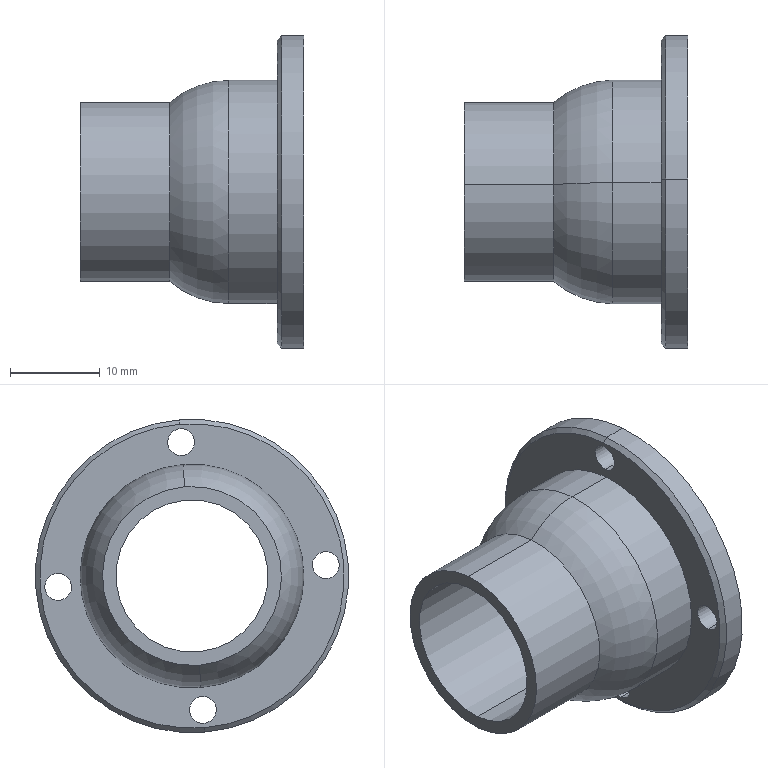Component | SolidWorks | 2-1 | 1 solid | 23 faces | box 25 x 35 x 35 mm | volume 5761 mm3 | cylinder 16 | plane 3 | torus 2 | cone 2 | commonest cylinder face diameters 3 x8 35 x2 17 x2 20 x2 25 x2
STEP:
#1=COLOUR_RGB('',0.7922,0.8196,0.9333);
#2=FILL_AREA_STYLE_COLOUR('',#1);
#3=FILL_AREA_STYLE('',(#2));
#4=SURFACE_STYLE_FILL_AREA(#3);
#5=SURFACE_SIDE_STYLE('',(#4));
#6=SURFACE_STYLE_USAGE(.BOTH.,#5);
#7=PRESENTATION_STYLE_ASSIGNMENT((#6));
#8=CARTESIAN_POINT('',(1.1,0.296,-0.4905));
#9=VERTEX_POINT('',#8);
#10=CARTESIAN_POINT('',(1.1,0.376,0.4905));
#11=VERTEX_POINT('',#10);
#12=CARTESIAN_POINT('',(1.1,0.336,0.));
#13=DIRECTION('',(1.,0.,0.));
#14=DIRECTION('',(0.,0.08123,0.9967));
#15=AXIS2_PLACEMENT_3D('',#12,#13,#14);
#16=CIRCLE('',#15,0.4921);
#17=EDGE_CURVE('',#9,#11,#16,.T.);
#18=ORIENTED_EDGE('',*,*,#17,.F.);
#19=CARTESIAN_POINT('',(0.8397,0.304,-0.3924));
#20=VERTEX_POINT('',#19);
#21=CARTESIAN_POINT('',(1.1,0.328,-0.0981));
#22=DIRECTION('',(0.,0.9967,-0.08123));
#23=DIRECTION('',(0.,0.08123,0.9967));
#24=AXIS2_PLACEMENT_3D('',#21,#22,#23);
#25=CIRCLE('',#24,0.3937);
#26=EDGE_CURVE('',#9,#20,#25,.T.);
#27=ORIENTED_EDGE('',*,*,#26,.T.);
#28=CARTESIAN_POINT('',(0.8397,0.368,0.3924));
#29=VERTEX_POINT('',#28);
#30=CARTESIAN_POINT('',(0.8397,0.336,0.));
#31=DIRECTION('',(1.,0.,0.));
#32=DIRECTION('',(0.,-0.08123,-0.9967));
#33=AXIS2_PLACEMENT_3D('',#30,#31,#32);
#34=CIRCLE('',#33,0.3937);
#35=EDGE_CURVE('',#20,#29,#34,.T.);
#36=ORIENTED_EDGE('',*,*,#35,.T.);
#37=CARTESIAN_POINT('',(1.1,0.344,0.0981));
#38=DIRECTION('',(0.,-0.9967,0.08123));
#39=DIRECTION('',(0.,-0.08123,-0.9967));
#40=AXIS2_PLACEMENT_3D('',#37,#38,#39);
#41=CIRCLE('',#40,0.3937);
#42=EDGE_CURVE('',#11,#29,#41,.T.);
#43=ORIENTED_EDGE('',*,*,#42,.F.);
#44=EDGE_LOOP('',(#18,#27,#36,#43));
#45=FACE_OUTER_BOUND('',#44,.T.);
#46=CARTESIAN_POINT('',(1.1,0.336,0.));
#47=DIRECTION('',(-1.,0.,0.));
#48=DIRECTION('',(0.,0.08123,0.9967));
#49=AXIS2_PLACEMENT_3D('',#46,#47,#48);
#50=TOROIDAL_SURFACE('',#49,0.09843,0.3937);
#51=ADVANCED_FACE('',(#45),#50,.T.);
#52=CARTESIAN_POINT('',(1.312,0.3904,0.6671));
#53=VERTEX_POINT('',#52);
#54=CARTESIAN_POINT('',(1.312,0.2816,-0.6671));
#55=VERTEX_POINT('',#54);
#56=CARTESIAN_POINT('',(1.312,0.336,0.));
#57=DIRECTION('',(-1.,0.,0.));
#58=DIRECTION('',(0.,-0.08123,-0.9967));
#59=AXIS2_PLACEMENT_3D('',#56,#57,#58);
#60=CIRCLE('',#59,0.6693);
#61=EDGE_CURVE('',#53,#55,#60,.T.);
#62=ORIENTED_EDGE('',*,*,#61,.F.);
#63=CARTESIAN_POINT('',(1.332,0.392,0.6867));
#64=VERTEX_POINT('',#63);
#65=CARTESIAN_POINT('',(1.332,0.392,0.6867));
#66=DIRECTION('',(0.7071,0.05744,0.7048));
#67=VECTOR('',#66,39.37);
#68=LINE('',#65,#67);
#69=EDGE_CURVE('',#53,#64,#68,.T.);
#70=ORIENTED_EDGE('',*,*,#69,.T.);
#71=CARTESIAN_POINT('',(1.332,0.28,-0.6867));
#72=VERTEX_POINT('',#71);
#73=CARTESIAN_POINT('',(1.332,0.336,0.));
#74=DIRECTION('',(1.,0.,0.));
#75=DIRECTION('',(0.,-0.08123,-0.9967));
#76=AXIS2_PLACEMENT_3D('',#73,#74,#75);
#77=CIRCLE('',#76,0.689);
#78=EDGE_CURVE('',#72,#64,#77,.T.);
#79=ORIENTED_EDGE('',*,*,#78,.F.);
#80=CARTESIAN_POINT('',(1.332,0.28,-0.6867));
#81=DIRECTION('',(0.7071,-0.05744,-0.7048));
#82=VECTOR('',#81,39.37);
#83=LINE('',#80,#82);
#84=EDGE_CURVE('',#55,#72,#83,.T.);
#85=ORIENTED_EDGE('',*,*,#84,.F.);
#86=EDGE_LOOP('',(#62,#70,#79,#85));
#87=FACE_OUTER_BOUND('',#86,.T.);
#88=CARTESIAN_POINT('',(1.332,0.336,0.));
#89=DIRECTION('',(1.,0.,0.));
#90=DIRECTION('',(0.,-0.08123,-0.9967));
#91=AXIS2_PLACEMENT_3D('',#88,#89,#90);
#92=CONICAL_SURFACE('',#91,0.689,0.7854);
#93=ADVANCED_FACE('',(#87),#92,.T.);
#94=CARTESIAN_POINT('',(1.43,0.2832,-0.6475));
#95=VERTEX_POINT('',#94);
#96=CARTESIAN_POINT('',(1.43,0.2928,-0.5297));
#97=VERTEX_POINT('',#96);
#98=CARTESIAN_POINT('',(1.43,0.288,-0.5886));
#99=DIRECTION('',(-1.,0.,0.));
#100=DIRECTION('',(0.,0.08123,0.9967));
#101=AXIS2_PLACEMENT_3D('',#98,#99,#100);
#102=CIRCLE('',#101,0.05906);
#103=EDGE_CURVE('',#95,#97,#102,.T.);
#104=ORIENTED_EDGE('',*,*,#103,.F.);
#105=CARTESIAN_POINT('',(1.312,0.2832,-0.6475));
#106=VERTEX_POINT('',#105);
#107=CARTESIAN_POINT('',(1.43,0.2832,-0.6475));
#108=DIRECTION('',(-1.,0.,0.));
#109=VECTOR('',#108,39.37);
#110=LINE('',#107,#109);
#111=EDGE_CURVE('',#95,#106,#110,.T.);
#112=ORIENTED_EDGE('',*,*,#111,.T.);
#113=CARTESIAN_POINT('',(1.312,0.2928,-0.5297));
#114=VERTEX_POINT('',#113);
#115=CARTESIAN_POINT('',(1.312,0.288,-0.5886));
#116=DIRECTION('',(-1.,0.,0.));
#117=DIRECTION('',(0.,0.08123,0.9967));
#118=AXIS2_PLACEMENT_3D('',#115,#116,#117);
#119=CIRCLE('',#118,0.05906);
#120=EDGE_CURVE('',#106,#114,#119,.T.);
#121=ORIENTED_EDGE('',*,*,#120,.T.);
#122=CARTESIAN_POINT('',(1.43,0.2928,-0.5297));
#123=DIRECTION('',(-1.,0.,0.));
#124=VECTOR('',#123,39.37);
#125=LINE('',#122,#124);
#126=EDGE_CURVE('',#97,#114,#125,.T.);
#127=ORIENTED_EDGE('',*,*,#126,.F.);
#128=EDGE_LOOP('',(#104,#112,#121,#127));
#129=FACE_OUTER_BOUND('',#128,.T.);
#130=CARTESIAN_POINT('',(1.43,0.288,-0.5886));
#131=DIRECTION('',(-1.,0.,0.));
#132=DIRECTION('',(0.,0.08123,0.9967));
#133=AXIS2_PLACEMENT_3D('',#130,#131,#132);
#134=CYLINDRICAL_SURFACE('',#133,0.05906);
#135=ADVANCED_FACE('',(#129),#134,.F.);
#136=CARTESIAN_POINT('',(1.43,-0.2574,-0.01089));
#137=VERTEX_POINT('',#136);
#138=CARTESIAN_POINT('',(1.43,-0.2478,0.1068));
#139=VERTEX_POINT('',#138);
#140=CARTESIAN_POINT('',(1.43,-0.2526,0.04797));
#141=DIRECTION('',(-1.,0.,0.));
#142=DIRECTION('',(0.,0.08123,0.9967));
#143=AXIS2_PLACEMENT_3D('',#140,#141,#142);
#144=CIRCLE('',#143,0.05906);
#145=EDGE_CURVE('',#137,#139,#144,.T.);
#146=ORIENTED_EDGE('',*,*,#145,.F.);
#147=CARTESIAN_POINT('',(1.312,-0.2574,-0.01089));
#148=VERTEX_POINT('',#147);
#149=CARTESIAN_POINT('',(1.43,-0.2574,-0.01089));
#150=DIRECTION('',(-1.,0.,0.));
#151=VECTOR('',#150,39.37);
#152=LINE('',#149,#151);
#153=EDGE_CURVE('',#137,#148,#152,.T.);
#154=ORIENTED_EDGE('',*,*,#153,.T.);
#155=CARTESIAN_POINT('',(1.312,-0.2478,0.1068));
#156=VERTEX_POINT('',#155);
#157=CARTESIAN_POINT('',(1.312,-0.2526,0.04797));
#158=DIRECTION('',(-1.,0.,0.));
#159=DIRECTION('',(0.,0.08123,0.9967));
#160=AXIS2_PLACEMENT_3D('',#157,#158,#159);
#161=CIRCLE('',#160,0.05906);
#162=EDGE_CURVE('',#148,#156,#161,.T.);
#163=ORIENTED_EDGE('',*,*,#162,.T.);
#164=CARTESIAN_POINT('',(1.43,-0.2478,0.1068));
#165=DIRECTION('',(-1.,0.,0.));
#166=VECTOR('',#165,39.37);
#167=LINE('',#164,#166);
#168=EDGE_CURVE('',#139,#156,#167,.T.);
#169=ORIENTED_EDGE('',*,*,#168,.F.);
#170=EDGE_LOOP('',(#146,#154,#163,#169));
#171=FACE_OUTER_BOUND('',#170,.T.);
#172=CARTESIAN_POINT('',(1.43,-0.2526,0.04797));
#173=DIRECTION('',(-1.,0.,0.));
#174=DIRECTION('',(0.,0.08123,0.9967));
#175=AXIS2_PLACEMENT_3D('',#172,#173,#174);
#176=CYLINDRICAL_SURFACE('',#175,0.05906);
#177=ADVANCED_FACE('',(#171),#176,.F.);
#178=CARTESIAN_POINT('',(1.43,0.3792,0.5297));
#179=VERTEX_POINT('',#178);
#180=CARTESIAN_POINT('',(1.43,0.3888,0.6475));
#181=VERTEX_POINT('',#180);
#182=CARTESIAN_POINT('',(1.43,0.384,0.5886));
#183=DIRECTION('',(-1.,0.,0.));
#184=DIRECTION('',(0.,0.08123,0.9967));
#185=AXIS2_PLACEMENT_3D('',#182,#183,#184);
#186=CIRCLE('',#185,0.05906);
#187=EDGE_CURVE('',#179,#181,#186,.T.);
#188=ORIENTED_EDGE('',*,*,#187,.F.);
#189=CARTESIAN_POINT('',(1.312,0.3792,0.5297));
#190=VERTEX_POINT('',#189);
#191=CARTESIAN_POINT('',(1.43,0.3792,0.5297));
#192=DIRECTION('',(-1.,0.,0.));
#193=VECTOR('',#192,39.37);
#194=LINE('',#191,#193);
#195=EDGE_CURVE('',#179,#190,#194,.T.);
#196=ORIENTED_EDGE('',*,*,#195,.T.);
#197=CARTESIAN_POINT('',(1.312,0.3888,0.6475));
#198=VERTEX_POINT('',#197);
#199=CARTESIAN_POINT('',(1.312,0.384,0.5886));
#200=DIRECTION('',(-1.,0.,0.));
#201=DIRECTION('',(0.,0.08123,0.9967));
#202=AXIS2_PLACEMENT_3D('',#199,#200,#201);
#203=CIRCLE('',#202,0.05906);
#204=EDGE_CURVE('',#190,#198,#203,.T.);
#205=ORIENTED_EDGE('',*,*,#204,.T.);
#206=CARTESIAN_POINT('',(1.43,0.3888,0.6475));
#207=DIRECTION('',(-1.,0.,0.));
#208=VECTOR('',#207,39.37);
#209=LINE('',#206,#208);
#210=EDGE_CURVE('',#181,#198,#209,.T.);
#211=ORIENTED_EDGE('',*,*,#210,.F.);
#212=EDGE_LOOP('',(#188,#196,#205,#211));
#213=FACE_OUTER_BOUND('',#212,.T.);
#214=CARTESIAN_POINT('',(1.43,0.384,0.5886));
#215=DIRECTION('',(-1.,0.,0.));
#216=DIRECTION('',(0.,0.08123,0.9967));
#217=AXIS2_PLACEMENT_3D('',#214,#215,#216);
#218=CYLINDRICAL_SURFACE('',#217,0.05906);
#219=ADVANCED_FACE('',(#213),#218,.F.);
#220=CARTESIAN_POINT('',(1.43,0.9198,-0.1068));
#221=VERTEX_POINT('',#220);
#222=CARTESIAN_POINT('',(1.43,0.9294,0.01089));
#223=VERTEX_POINT('',#222);
#224=CARTESIAN_POINT('',(1.43,0.9246,-0.04797));
#225=DIRECTION('',(-1.,0.,0.));
#226=DIRECTION('',(0.,0.08123,0.9967));
#227=AXIS2_PLACEMENT_3D('',#224,#225,#226);
#228=CIRCLE('',#227,0.05906);
#229=EDGE_CURVE('',#221,#223,#228,.T.);
#230=ORIENTED_EDGE('',*,*,#229,.F.);
#231=CARTESIAN_POINT('',(1.312,0.9198,-0.1068));
#232=VERTEX_POINT('',#231);
#233=CARTESIAN_POINT('',(1.43,0.9198,-0.1068));
#234=DIRECTION('',(-1.,0.,0.));
#235=VECTOR('',#234,39.37);
#236=LINE('',#233,#235);
#237=EDGE_CURVE('',#221,#232,#236,.T.);
#238=ORIENTED_EDGE('',*,*,#237,.T.);
#239=CARTESIAN_POINT('',(1.312,0.9294,0.01089));
#240=VERTEX_POINT('',#239);
#241=CARTESIAN_POINT('',(1.312,0.9246,-0.04797));
#242=DIRECTION('',(-1.,0.,0.));
#243=DIRECTION('',(0.,0.08123,0.9967));
#244=AXIS2_PLACEMENT_3D('',#241,#242,#243);
#245=CIRCLE('',#244,0.05906);
#246=EDGE_CURVE('',#232,#240,#245,.T.);
#247=ORIENTED_EDGE('',*,*,#246,.T.);
#248=CARTESIAN_POINT('',(1.43,0.9294,0.01089));
#249=DIRECTION('',(-1.,0.,0.));
#250=VECTOR('',#249,39.37);
#251=LINE('',#248,#250);
#252=EDGE_CURVE('',#223,#240,#251,.T.);
#253=ORIENTED_EDGE('',*,*,#252,.F.);
#254=EDGE_LOOP('',(#230,#238,#247,#253));
#255=FACE_OUTER_BOUND('',#254,.T.);
#256=CARTESIAN_POINT('',(1.43,0.9246,-0.04797));
#257=DIRECTION('',(-1.,0.,0.));
#258=DIRECTION('',(0.,0.08123,0.9967));
#259=AXIS2_PLACEMENT_3D('',#256,#257,#258);
#260=CYLINDRICAL_SURFACE('',#259,0.05906);
#261=ADVANCED_FACE('',(#255),#260,.F.);
#262=ORIENTED_EDGE('',*,*,#78,.T.);
#263=CARTESIAN_POINT('',(1.43,0.392,0.6867));
#264=VERTEX_POINT('',#263);
#265=CARTESIAN_POINT('',(1.312,0.392,0.6867));
#266=DIRECTION('',(1.,0.,0.));
#267=VECTOR('',#266,39.37);
#268=LINE('',#265,#267);
#269=EDGE_CURVE('',#64,#264,#268,.T.);
#270=ORIENTED_EDGE('',*,*,#269,.T.);
#271=CARTESIAN_POINT('',(1.43,0.28,-0.6867));
#272=VERTEX_POINT('',#271);
#273=CARTESIAN_POINT('',(1.43,0.336,0.));
#274=DIRECTION('',(1.,0.,0.));
#275=DIRECTION('',(0.,-0.08123,-0.9967));
#276=AXIS2_PLACEMENT_3D('',#273,#274,#275);
#277=CIRCLE('',#276,0.689);
#278=EDGE_CURVE('',#272,#264,#277,.T.);
#279=ORIENTED_EDGE('',*,*,#278,.F.);
#280=CARTESIAN_POINT('',(1.312,0.28,-0.6867));
#281=DIRECTION('',(1.,0.,0.));
#282=VECTOR('',#281,39.37);
#283=LINE('',#280,#282);
#284=EDGE_CURVE('',#72,#272,#283,.T.);
#285=ORIENTED_EDGE('',*,*,#284,.F.);
#286=EDGE_LOOP('',(#262,#270,#279,#285));
#287=FACE_OUTER_BOUND('',#286,.T.);
#288=CARTESIAN_POINT('',(1.312,0.336,0.));
#289=DIRECTION('',(1.,0.,0.));
#290=DIRECTION('',(0.,-0.08123,-0.9967));
#291=AXIS2_PLACEMENT_3D('',#288,#289,#290);
#292=CYLINDRICAL_SURFACE('',#291,0.689);
#293=ADVANCED_FACE('',(#287),#292,.T.);
#294=CARTESIAN_POINT('',(1.43,0.3632,0.3335));
#295=VERTEX_POINT('',#294);
#296=CARTESIAN_POINT('',(1.43,0.3088,-0.3335));
#297=VERTEX_POINT('',#296);
#298=CARTESIAN_POINT('',(1.43,0.336,0.));
#299=DIRECTION('',(1.,0.,0.));
#300=DIRECTION('',(0.,-0.08123,-0.9967));
#301=AXIS2_PLACEMENT_3D('',#298,#299,#300);
#302=CIRCLE('',#301,0.3346);
#303=EDGE_CURVE('',#295,#297,#302,.T.);
#304=ORIENTED_EDGE('',*,*,#303,.T.);
#305=CARTESIAN_POINT('',(0.446,0.3088,-0.3335));
#306=VERTEX_POINT('',#305);
#307=CARTESIAN_POINT('',(0.8397,0.3088,-0.3335));
#308=DIRECTION('',(-1.,0.,0.));
#309=VECTOR('',#308,39.37);
#310=LINE('',#307,#309);
#311=EDGE_CURVE('',#297,#306,#310,.T.);
#312=ORIENTED_EDGE('',*,*,#311,.T.);
#313=CARTESIAN_POINT('',(0.446,0.3632,0.3335));
#314=VERTEX_POINT('',#313);
#315=CARTESIAN_POINT('',(0.446,0.336,0.));
#316=DIRECTION('',(1.,0.,0.));
#317=DIRECTION('',(0.,-0.08123,-0.9967));
#318=AXIS2_PLACEMENT_3D('',#315,#316,#317);
#319=CIRCLE('',#318,0.3346);
#320=EDGE_CURVE('',#314,#306,#319,.T.);
#321=ORIENTED_EDGE('',*,*,#320,.F.);
#322=CARTESIAN_POINT('',(0.8397,0.3632,0.3335));
#323=DIRECTION('',(-1.,0.,0.));
#324=VECTOR('',#323,39.37);
#325=LINE('',#322,#324);
#326=EDGE_CURVE('',#295,#314,#325,.T.);
#327=ORIENTED_EDGE('',*,*,#326,.F.);
#328=EDGE_LOOP('',(#304,#312,#321,#327));
#329=FACE_OUTER_BOUND('',#328,.T.);
#330=CARTESIAN_POINT('',(0.8397,0.336,0.));
#331=DIRECTION('',(-1.,0.,0.));
#332=DIRECTION('',(0.,0.08123,0.9967));
#333=AXIS2_PLACEMENT_3D('',#330,#331,#332);
#334=CYLINDRICAL_SURFACE('',#333,0.3346);
#335=ADVANCED_FACE('',(#329),#334,.F.);
#336=ORIENTED_EDGE('',*,*,#35,.F.);
#337=CARTESIAN_POINT('',(0.446,0.304,-0.3924));
#338=VERTEX_POINT('',#337);
#339=CARTESIAN_POINT('',(0.8397,0.304,-0.3924));
#340=DIRECTION('',(-1.,0.,0.));
#341=VECTOR('',#340,39.37);
#342=LINE('',#339,#341);
#343=EDGE_CURVE('',#20,#338,#342,.T.);
#344=ORIENTED_EDGE('',*,*,#343,.T.);
#345=CARTESIAN_POINT('',(0.446,0.368,0.3924));
#346=VERTEX_POINT('',#345);
#347=CARTESIAN_POINT('',(0.446,0.336,0.));
#348=DIRECTION('',(1.,0.,0.));
#349=DIRECTION('',(0.,-0.08123,-0.9967));
#350=AXIS2_PLACEMENT_3D('',#347,#348,#349);
#351=CIRCLE('',#350,0.3937);
#352=EDGE_CURVE('',#338,#346,#351,.T.);
#353=ORIENTED_EDGE('',*,*,#352,.T.);
#354=CARTESIAN_POINT('',(0.8397,0.368,0.3924));
#355=DIRECTION('',(-1.,0.,0.));
#356=VECTOR('',#355,39.37);
#357=LINE('',#354,#356);
#358=EDGE_CURVE('',#29,#346,#357,.T.);
#359=ORIENTED_EDGE('',*,*,#358,.F.);
#360=EDGE_LOOP('',(#336,#344,#353,#359));
#361=FACE_OUTER_BOUND('',#360,.T.);
#362=CARTESIAN_POINT('',(0.8397,0.336,0.));
#363=DIRECTION('',(-1.,0.,0.));
#364=DIRECTION('',(0.,0.08123,0.9967));
#365=AXIS2_PLACEMENT_3D('',#362,#363,#364);
#366=CYLINDRICAL_SURFACE('',#365,0.3937);
#367=ADVANCED_FACE('',(#361),#366,.T.);
#368=CARTESIAN_POINT('',(1.312,0.296,-0.4905));
#369=VERTEX_POINT('',#368);
#370=CARTESIAN_POINT('',(1.312,0.376,0.4905));
#371=VERTEX_POINT('',#370);
#372=CARTESIAN_POINT('',(1.312,0.336,0.));
#373=DIRECTION('',(1.,0.,0.));
#374=DIRECTION('',(0.,-0.08123,-0.9967));
#375=AXIS2_PLACEMENT_3D('',#372,#373,#374);
#376=CIRCLE('',#375,0.4921);
#377=EDGE_CURVE('',#369,#371,#376,.T.);
#378=ORIENTED_EDGE('',*,*,#377,.F.);
#379=CARTESIAN_POINT('',(1.43,0.296,-0.4905));
#380=DIRECTION('',(-1.,0.,0.));
#381=VECTOR('',#380,39.37);
#382=LINE('',#379,#381);
#383=EDGE_CURVE('',#369,#9,#382,.T.);
#384=ORIENTED_EDGE('',*,*,#383,.T.);
#385=ORIENTED_EDGE('',*,*,#17,.T.);
#386=CARTESIAN_POINT('',(1.43,0.376,0.4905));
#387=DIRECTION('',(-1.,0.,0.));
#388=VECTOR('',#387,39.37);
#389=LINE('',#386,#388);
#390=EDGE_CURVE('',#371,#11,#389,.T.);
#391=ORIENTED_EDGE('',*,*,#390,.F.);
#392=EDGE_LOOP('',(#378,#384,#385,#391));
#393=FACE_OUTER_BOUND('',#392,.T.);
#394=CARTESIAN_POINT('',(1.43,0.336,0.));
#395=DIRECTION('',(-1.,0.,0.));
#396=DIRECTION('',(0.,0.08123,0.9967));
#397=AXIS2_PLACEMENT_3D('',#394,#395,#396);
#398=CYLINDRICAL_SURFACE('',#397,0.4921);
#399=ADVANCED_FACE('',(#393),#398,.T.);
#400=ORIENTED_EDGE('',*,*,#383,.F.);
#401=CARTESIAN_POINT('',(1.312,0.336,0.));
#402=DIRECTION('',(1.,0.,0.));
#403=DIRECTION('',(0.,-0.08123,-0.9967));
#404=AXIS2_PLACEMENT_3D('',#401,#402,#403);
#405=CIRCLE('',#404,0.4921);
#406=EDGE_CURVE('',#371,#369,#405,.T.);
#407=ORIENTED_EDGE('',*,*,#406,.F.);
#408=ORIENTED_EDGE('',*,*,#390,.T.);
#409=CARTESIAN_POINT('',(1.1,0.336,0.));
#410=DIRECTION('',(1.,0.,0.));
#411=DIRECTION('',(0.,0.08123,0.9967));
#412=AXIS2_PLACEMENT_3D('',#409,#410,#411);
#413=CIRCLE('',#412,0.4921);
#414=EDGE_CURVE('',#11,#9,#413,.T.);
#415=ORIENTED_EDGE('',*,*,#414,.T.);
#416=EDGE_LOOP('',(#400,#407,#408,#415));
#417=FACE_OUTER_BOUND('',#416,.T.);
#418=CARTESIAN_POINT('',(1.43,0.336,0.));
#419=DIRECTION('',(-1.,0.,0.));
#420=DIRECTION('',(0.,0.08123,0.9967));
#421=AXIS2_PLACEMENT_3D('',#418,#419,#420);
#422=CYLINDRICAL_SURFACE('',#421,0.4921);
#423=ADVANCED_FACE('',(#417),#422,.T.);
#424=CARTESIAN_POINT('',(0.446,0.336,0.));
#425=DIRECTION('',(1.,0.,0.));
#426=DIRECTION('',(0.,-0.08123,-0.9967));
#427=AXIS2_PLACEMENT_3D('',#424,#425,#426);
#428=CIRCLE('',#427,0.3937);
#429=EDGE_CURVE('',#346,#338,#428,.T.);
#430=ORIENTED_EDGE('',*,*,#429,.F.);
#431=ORIENTED_EDGE('',*,*,#352,.F.);
#432=EDGE_LOOP('',(#430,#431));
#433=FACE_OUTER_BOUND('',#432,.T.);
#434=ORIENTED_EDGE('',*,*,#320,.T.);
#435=CARTESIAN_POINT('',(0.446,0.336,0.));
#436=DIRECTION('',(1.,0.,0.));
#437=DIRECTION('',(0.,-0.08123,-0.9967));
#438=AXIS2_PLACEMENT_3D('',#435,#436,#437);
#439=CIRCLE('',#438,0.3346);
#440=EDGE_CURVE('',#306,#314,#439,.T.);
#441=ORIENTED_EDGE('',*,*,#440,.T.);
#442=EDGE_LOOP('',(#434,#441));
#443=FACE_BOUND('',#442,.T.);
#444=CARTESIAN_POINT('',(0.446,0.336,0.));
#445=DIRECTION('',(1.,0.,0.));
#446=DIRECTION('',(0.,-0.08123,-0.9967));
#447=AXIS2_PLACEMENT_3D('',#444,#445,#446);
#448=PLANE('',#447);
#449=ADVANCED_FACE('',(#433,#443),#448,.F.);
#450=ORIENTED_EDGE('',*,*,#343,.F.);
#451=CARTESIAN_POINT('',(0.8397,0.336,0.));
#452=DIRECTION('',(1.,0.,0.));
#453=DIRECTION('',(0.,-0.08123,-0.9967));
#454=AXIS2_PLACEMENT_3D('',#451,#452,#453);
#455=CIRCLE('',#454,0.3937);
#456=EDGE_CURVE('',#29,#20,#455,.T.);
#457=ORIENTED_EDGE('',*,*,#456,.F.);
#458=ORIENTED_EDGE('',*,*,#358,.T.);
#459=ORIENTED_EDGE('',*,*,#429,.T.);
#460=EDGE_LOOP('',(#450,#457,#458,#459));
#461=FACE_OUTER_BOUND('',#460,.T.);
#462=CARTESIAN_POINT('',(0.8397,0.336,0.));
#463=DIRECTION('',(-1.,0.,0.));
#464=DIRECTION('',(0.,0.08123,0.9967));
#465=AXIS2_PLACEMENT_3D('',#462,#463,#464);
#466=CYLINDRICAL_SURFACE('',#465,0.3937);
#467=ADVANCED_FACE('',(#461),#466,.T.);
#468=ORIENTED_EDGE('',*,*,#311,.F.);
#469=CARTESIAN_POINT('',(1.43,0.336,0.));
#470=DIRECTION('',(1.,0.,0.));
#471=DIRECTION('',(0.,-0.08123,-0.9967));
#472=AXIS2_PLACEMENT_3D('',#469,#470,#471);
#473=CIRCLE('',#472,0.3346);
#474=EDGE_CURVE('',#297,#295,#473,.T.);
#475=ORIENTED_EDGE('',*,*,#474,.T.);
#476=ORIENTED_EDGE('',*,*,#326,.T.);
#477=ORIENTED_EDGE('',*,*,#440,.F.);
#478=EDGE_LOOP('',(#468,#475,#476,#477));
#479=FACE_OUTER_BOUND('',#478,.T.);
#480=CARTESIAN_POINT('',(0.8397,0.336,0.));
#481=DIRECTION('',(-1.,0.,0.));
#482=DIRECTION('',(0.,0.08123,0.9967));
#483=AXIS2_PLACEMENT_3D('',#480,#481,#482);
#484=CYLINDRICAL_SURFACE('',#483,0.3346);
#485=ADVANCED_FACE('',(#479),#484,.F.);
#486=CARTESIAN_POINT('',(1.43,0.288,-0.5886));
#487=DIRECTION('',(-1.,0.,0.));
#488=DIRECTION('',(0.,0.08123,0.9967));
#489=AXIS2_PLACEMENT_3D('',#486,#487,#488);
#490=CIRCLE('',#489,0.05906);
#491=EDGE_CURVE('',#97,#95,#490,.T.);
#492=ORIENTED_EDGE('',*,*,#491,.T.);
#493=ORIENTED_EDGE('',*,*,#103,.T.);
#494=EDGE_LOOP('',(#492,#493));
#495=FACE_BOUND('',#494,.T.);
#496=CARTESIAN_POINT('',(1.43,-0.2526,0.04797));
#497=DIRECTION('',(-1.,0.,0.));
#498=DIRECTION('',(0.,0.08123,0.9967));
#499=AXIS2_PLACEMENT_3D('',#496,#497,#498);
#500=CIRCLE('',#499,0.05906);
#501=EDGE_CURVE('',#139,#137,#500,.T.);
#502=ORIENTED_EDGE('',*,*,#501,.T.);
#503=ORIENTED_EDGE('',*,*,#145,.T.);
#504=EDGE_LOOP('',(#502,#503));
#505=FACE_BOUND('',#504,.T.);
#506=CARTESIAN_POINT('',(1.43,0.384,0.5886));
#507=DIRECTION('',(-1.,0.,0.));
#508=DIRECTION('',(0.,0.08123,0.9967));
#509=AXIS2_PLACEMENT_3D('',#506,#507,#508);
#510=CIRCLE('',#509,0.05906);
#511=EDGE_CURVE('',#181,#179,#510,.T.);
#512=ORIENTED_EDGE('',*,*,#511,.T.);
#513=ORIENTED_EDGE('',*,*,#187,.T.);
#514=EDGE_LOOP('',(#512,#513));
#515=FACE_BOUND('',#514,.T.);
#516=CARTESIAN_POINT('',(1.43,0.9246,-0.04797));
#517=DIRECTION('',(-1.,0.,0.));
#518=DIRECTION('',(0.,0.08123,0.9967));
#519=AXIS2_PLACEMENT_3D('',#516,#517,#518);
#520=CIRCLE('',#519,0.05906);
#521=EDGE_CURVE('',#223,#221,#520,.T.);
#522=ORIENTED_EDGE('',*,*,#521,.T.);
#523=ORIENTED_EDGE('',*,*,#229,.T.);
#524=EDGE_LOOP('',(#522,#523));
#525=FACE_BOUND('',#524,.T.);
#526=ORIENTED_EDGE('',*,*,#303,.F.);
#527=ORIENTED_EDGE('',*,*,#474,.F.);
#528=EDGE_LOOP('',(#526,#527));
#529=FACE_BOUND('',#528,.T.);
#530=ORIENTED_EDGE('',*,*,#278,.T.);
#531=CARTESIAN_POINT('',(1.43,0.336,0.));
#532=DIRECTION('',(1.,0.,0.));
#533=DIRECTION('',(0.,-0.08123,-0.9967));
#534=AXIS2_PLACEMENT_3D('',#531,#532,#533);
#535=CIRCLE('',#534,0.689);
#536=EDGE_CURVE('',#264,#272,#535,.T.);
#537=ORIENTED_EDGE('',*,*,#536,.T.);
#538=EDGE_LOOP('',(#530,#537));
#539=FACE_OUTER_BOUND('',#538,.T.);
#540=CARTESIAN_POINT('',(1.43,0.336,0.));
#541=DIRECTION('',(1.,0.,0.));
#542=DIRECTION('',(0.,-0.08123,-0.9967));
#543=AXIS2_PLACEMENT_3D('',#540,#541,#542);
#544=PLANE('',#543);
#545=ADVANCED_FACE('',(#495,#505,#515,#525,#529,#539),#544,.T.);
#546=CARTESIAN_POINT('',(1.312,0.336,0.));
#547=DIRECTION('',(-1.,0.,0.));
#548=DIRECTION('',(0.,-0.08123,-0.9967));
#549=AXIS2_PLACEMENT_3D('',#546,#547,#548);
#550=CIRCLE('',#549,0.6693);
#551=EDGE_CURVE('',#55,#53,#550,.T.);
#552=ORIENTED_EDGE('',*,*,#551,.T.);
#553=ORIENTED_EDGE('',*,*,#61,.T.);
#554=EDGE_LOOP('',(#552,#553));
#555=FACE_OUTER_BOUND('',#554,.T.);
#556=CARTESIAN_POINT('',(1.312,0.288,-0.5886));
#557=DIRECTION('',(-1.,0.,0.));
#558=DIRECTION('',(0.,0.08123,0.9967));
#559=AXIS2_PLACEMENT_3D('',#556,#557,#558);
#560=CIRCLE('',#559,0.05906);
#561=EDGE_CURVE('',#114,#106,#560,.T.);
#562=ORIENTED_EDGE('',*,*,#561,.F.);
#563=ORIENTED_EDGE('',*,*,#120,.F.);
#564=EDGE_LOOP('',(#562,#563));
#565=FACE_BOUND('',#564,.T.);
#566=CARTESIAN_POINT('',(1.312,-0.2526,0.04797));
#567=DIRECTION('',(-1.,0.,0.));
#568=DIRECTION('',(0.,0.08123,0.9967));
#569=AXIS2_PLACEMENT_3D('',#566,#567,#568);
#570=CIRCLE('',#569,0.05906);
#571=EDGE_CURVE('',#156,#148,#570,.T.);
#572=ORIENTED_EDGE('',*,*,#571,.F.);
#573=ORIENTED_EDGE('',*,*,#162,.F.);
#574=EDGE_LOOP('',(#572,#573));
#575=FACE_BOUND('',#574,.T.);
#576=CARTESIAN_POINT('',(1.312,0.384,0.5886));
#577=DIRECTION('',(-1.,0.,0.));
#578=DIRECTION('',(0.,0.08123,0.9967));
#579=AXIS2_PLACEMENT_3D('',#576,#577,#578);
#580=CIRCLE('',#579,0.05906);
#581=EDGE_CURVE('',#198,#190,#580,.T.);
#582=ORIENTED_EDGE('',*,*,#581,.F.);
#583=ORIENTED_EDGE('',*,*,#204,.F.);
#584=EDGE_LOOP('',(#582,#583));
#585=FACE_BOUND('',#584,.T.);
#586=CARTESIAN_POINT('',(1.312,0.9246,-0.04797));
#587=DIRECTION('',(-1.,0.,0.));
#588=DIRECTION('',(0.,0.08123,0.9967));
#589=AXIS2_PLACEMENT_3D('',#586,#587,#588);
#590=CIRCLE('',#589,0.05906);
#591=EDGE_CURVE('',#240,#232,#590,.T.);
#592=ORIENTED_EDGE('',*,*,#591,.F.);
#593=ORIENTED_EDGE('',*,*,#246,.F.);
#594=EDGE_LOOP('',(#592,#593));
#595=FACE_BOUND('',#594,.T.);
#596=ORIENTED_EDGE('',*,*,#406,.T.);
#597=ORIENTED_EDGE('',*,*,#377,.T.);
#598=EDGE_LOOP('',(#596,#597));
#599=FACE_BOUND('',#598,.T.);
#600=CARTESIAN_POINT('',(1.312,0.336,0.));
#601=DIRECTION('',(1.,0.,0.));
#602=DIRECTION('',(0.,-0.08123,-0.9967));
#603=AXIS2_PLACEMENT_3D('',#600,#601,#602);
#604=PLANE('',#603);
#605=ADVANCED_FACE('',(#555,#565,#575,#585,#595,#599),#604,.F.);
#606=ORIENTED_EDGE('',*,*,#269,.F.);
#607=CARTESIAN_POINT('',(1.332,0.336,0.));
#608=DIRECTION('',(1.,0.,0.));
#609=DIRECTION('',(0.,-0.08123,-0.9967));
#610=AXIS2_PLACEMENT_3D('',#607,#608,#609);
#611=CIRCLE('',#610,0.689);
#612=EDGE_CURVE('',#64,#72,#611,.T.);
#613=ORIENTED_EDGE('',*,*,#612,.T.);
#614=ORIENTED_EDGE('',*,*,#284,.T.);
#615=ORIENTED_EDGE('',*,*,#536,.F.);
#616=EDGE_LOOP('',(#606,#613,#614,#615));
#617=FACE_OUTER_BOUND('',#616,.T.);
#618=CARTESIAN_POINT('',(1.312,0.336,0.));
#619=DIRECTION('',(1.,0.,0.));
#620=DIRECTION('',(0.,-0.08123,-0.9967));
#621=AXIS2_PLACEMENT_3D('',#618,#619,#620);
#622=CYLINDRICAL_SURFACE('',#621,0.689);
#623=ADVANCED_FACE('',(#617),#622,.T.);
#624=ORIENTED_EDGE('',*,*,#237,.F.);
#625=ORIENTED_EDGE('',*,*,#521,.F.);
#626=ORIENTED_EDGE('',*,*,#252,.T.);
#627=ORIENTED_EDGE('',*,*,#591,.T.);
#628=EDGE_LOOP('',(#624,#625,#626,#627));
#629=FACE_OUTER_BOUND('',#628,.T.);
#630=CARTESIAN_POINT('',(1.43,0.9246,-0.04797));
#631=DIRECTION('',(-1.,0.,0.));
#632=DIRECTION('',(0.,0.08123,0.9967));
#633=AXIS2_PLACEMENT_3D('',#630,#631,#632);
#634=CYLINDRICAL_SURFACE('',#633,0.05906);
#635=ADVANCED_FACE('',(#629),#634,.F.);
#636=ORIENTED_EDGE('',*,*,#195,.F.);
#637=ORIENTED_EDGE('',*,*,#511,.F.);
#638=ORIENTED_EDGE('',*,*,#210,.T.);
#639=ORIENTED_EDGE('',*,*,#581,.T.);
#640=EDGE_LOOP('',(#636,#637,#638,#639));
#641=FACE_OUTER_BOUND('',#640,.T.);
#642=CARTESIAN_POINT('',(1.43,0.384,0.5886));
#643=DIRECTION('',(-1.,0.,0.));
#644=DIRECTION('',(0.,0.08123,0.9967));
#645=AXIS2_PLACEMENT_3D('',#642,#643,#644);
#646=CYLINDRICAL_SURFACE('',#645,0.05906);
#647=ADVANCED_FACE('',(#641),#646,.F.);
#648=ORIENTED_EDGE('',*,*,#153,.F.);
#649=ORIENTED_EDGE('',*,*,#501,.F.);
#650=ORIENTED_EDGE('',*,*,#168,.T.);
#651=ORIENTED_EDGE('',*,*,#571,.T.);
#652=EDGE_LOOP('',(#648,#649,#650,#651));
#653=FACE_OUTER_BOUND('',#652,.T.);
#654=CARTESIAN_POINT('',(1.43,-0.2526,0.04797));
#655=DIRECTION('',(-1.,0.,0.));
#656=DIRECTION('',(0.,0.08123,0.9967));
#657=AXIS2_PLACEMENT_3D('',#654,#655,#656);
#658=CYLINDRICAL_SURFACE('',#657,0.05906);
#659=ADVANCED_FACE('',(#653),#658,.F.);
#660=ORIENTED_EDGE('',*,*,#111,.F.);
#661=ORIENTED_EDGE('',*,*,#491,.F.);
#662=ORIENTED_EDGE('',*,*,#126,.T.);
#663=ORIENTED_EDGE('',*,*,#561,.T.);
#664=EDGE_LOOP('',(#660,#661,#662,#663));
#665=FACE_OUTER_BOUND('',#664,.T.);
#666=CARTESIAN_POINT('',(1.43,0.288,-0.5886));
#667=DIRECTION('',(-1.,0.,0.));
#668=DIRECTION('',(0.,0.08123,0.9967));
#669=AXIS2_PLACEMENT_3D('',#666,#667,#668);
#670=CYLINDRICAL_SURFACE('',#669,0.05906);
#671=ADVANCED_FACE('',(#665),#670,.F.);
#672=ORIENTED_EDGE('',*,*,#69,.F.);
#673=ORIENTED_EDGE('',*,*,#551,.F.);
#674=ORIENTED_EDGE('',*,*,#84,.T.);
#675=ORIENTED_EDGE('',*,*,#612,.F.);
#676=EDGE_LOOP('',(#672,#673,#674,#675));
#677=FACE_OUTER_BOUND('',#676,.T.);
#678=CARTESIAN_POINT('',(1.332,0.336,0.));
#679=DIRECTION('',(1.,0.,0.));
#680=DIRECTION('',(0.,-0.08123,-0.9967));
#681=AXIS2_PLACEMENT_3D('',#678,#679,#680);
#682=CONICAL_SURFACE('',#681,0.689,0.7854);
#683=ADVANCED_FACE('',(#677),#682,.T.);
#684=ORIENTED_EDGE('',*,*,#26,.F.);
#685=ORIENTED_EDGE('',*,*,#414,.F.);
#686=ORIENTED_EDGE('',*,*,#42,.T.);
#687=ORIENTED_EDGE('',*,*,#456,.T.);
#688=EDGE_LOOP('',(#684,#685,#686,#687));
#689=FACE_OUTER_BOUND('',#688,.T.);
#690=CARTESIAN_POINT('',(1.1,0.336,0.));
#691=DIRECTION('',(-1.,0.,0.));
#692=DIRECTION('',(0.,0.08123,0.9967));
#693=AXIS2_PLACEMENT_3D('',#690,#691,#692);
#694=TOROIDAL_SURFACE('',#693,0.09843,0.3937);
#695=ADVANCED_FACE('',(#689),#694,.T.);
#696=CLOSED_SHELL('',(#51,#93,#135,#177,#219,#261,#293,#335,#367,#399,#423,#449,#467,#485,#545,#605,#623,#635,#647,#659,#671,#683,#695));
#697=MANIFOLD_SOLID_BREP('',#696);
#698=STYLED_ITEM('',(#7),#697);
#699=PRESENTATION_LAYER_ASSIGNMENT('','',(#698));
#700=CARTESIAN_POINT('',(0.,0.,0.));
#701=DIRECTION('',(0.,0.,1.));
#702=DIRECTION('',(1.,0.,0.));
#703=AXIS2_PLACEMENT_3D('',#700,#701,#702);
#704=(LENGTH_UNIT()NAMED_UNIT(*)SI_UNIT($,.METRE.));
#705=LENGTH_MEASURE_WITH_UNIT(LENGTH_MEASURE(0.0254),#704);
#706=DIMENSIONAL_EXPONENTS(1.,0.,0.,0.,0.,0.,0.);
#707=(CONVERSION_BASED_UNIT('',#705)LENGTH_UNIT()NAMED_UNIT(#706));
#708=UNCERTAINTY_MEASURE_WITH_UNIT(LENGTH_MEASURE(0.00001),#707,'','');
#709=(NAMED_UNIT(*)PLANE_ANGLE_UNIT()SI_UNIT($,.RADIAN.));
#710=(NAMED_UNIT(*)SI_UNIT($,.STERADIAN.)SOLID_ANGLE_UNIT());
#711=(GEOMETRIC_REPRESENTATION_CONTEXT(3)GLOBAL_UNCERTAINTY_ASSIGNED_CONTEXT((#708))GLOBAL_UNIT_ASSIGNED_CONTEXT((#707,#709,#710))REPRESENTATION_CONTEXT('',''));
#712=ADVANCED_BREP_SHAPE_REPRESENTATION('',(#697,#703),#711);
#713=(LENGTH_UNIT()NAMED_UNIT(*)SI_UNIT($,.METRE.));
#714=LENGTH_MEASURE_WITH_UNIT(LENGTH_MEASURE(0.0254),#713);
#715=DIMENSIONAL_EXPONENTS(1.,0.,0.,0.,0.,0.,0.);
#716=(CONVERSION_BASED_UNIT('',#714)LENGTH_UNIT()NAMED_UNIT(#715));
#717=UNCERTAINTY_MEASURE_WITH_UNIT(LENGTH_MEASURE(0.00001),#716,'','');
#718=(NAMED_UNIT(*)PLANE_ANGLE_UNIT()SI_UNIT($,.RADIAN.));
#719=(NAMED_UNIT(*)SI_UNIT($,.STERADIAN.)SOLID_ANGLE_UNIT());
#720=(GEOMETRIC_REPRESENTATION_CONTEXT(3)GLOBAL_UNCERTAINTY_ASSIGNED_CONTEXT((#717))GLOBAL_UNIT_ASSIGNED_CONTEXT((#716,#718,#719))REPRESENTATION_CONTEXT('',''));
#721=MECHANICAL_DESIGN_GEOMETRIC_PRESENTATION_REPRESENTATION('',(#698),#720);